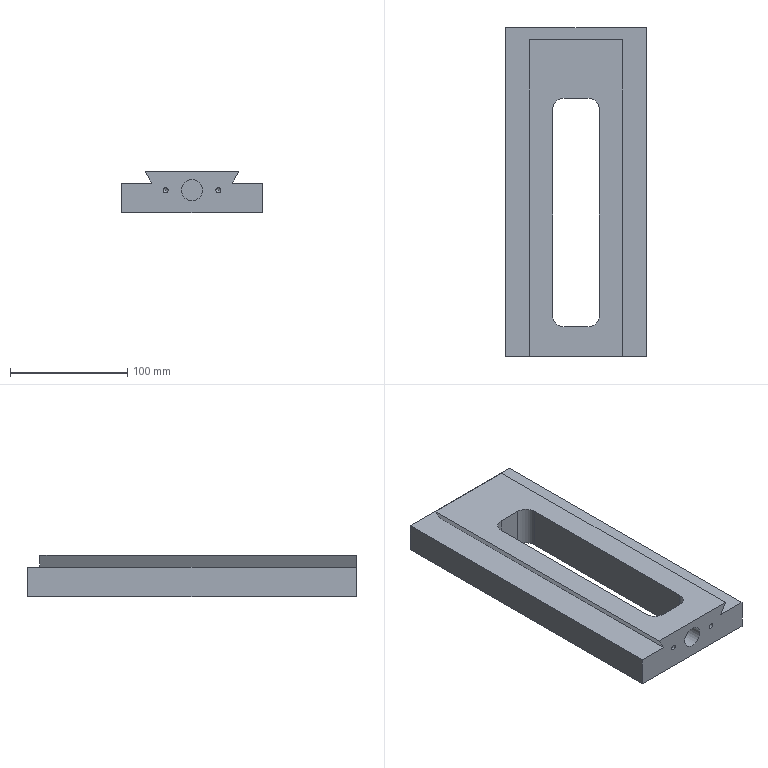Component | NX | SLIDE | 1 solid | 39 faces | volume 759740 mm3 | cylinder 15 | plane 14 | cone 10 | commonest cylinder face diameters 5 x8 20 x4 4.2 x2 18 x1